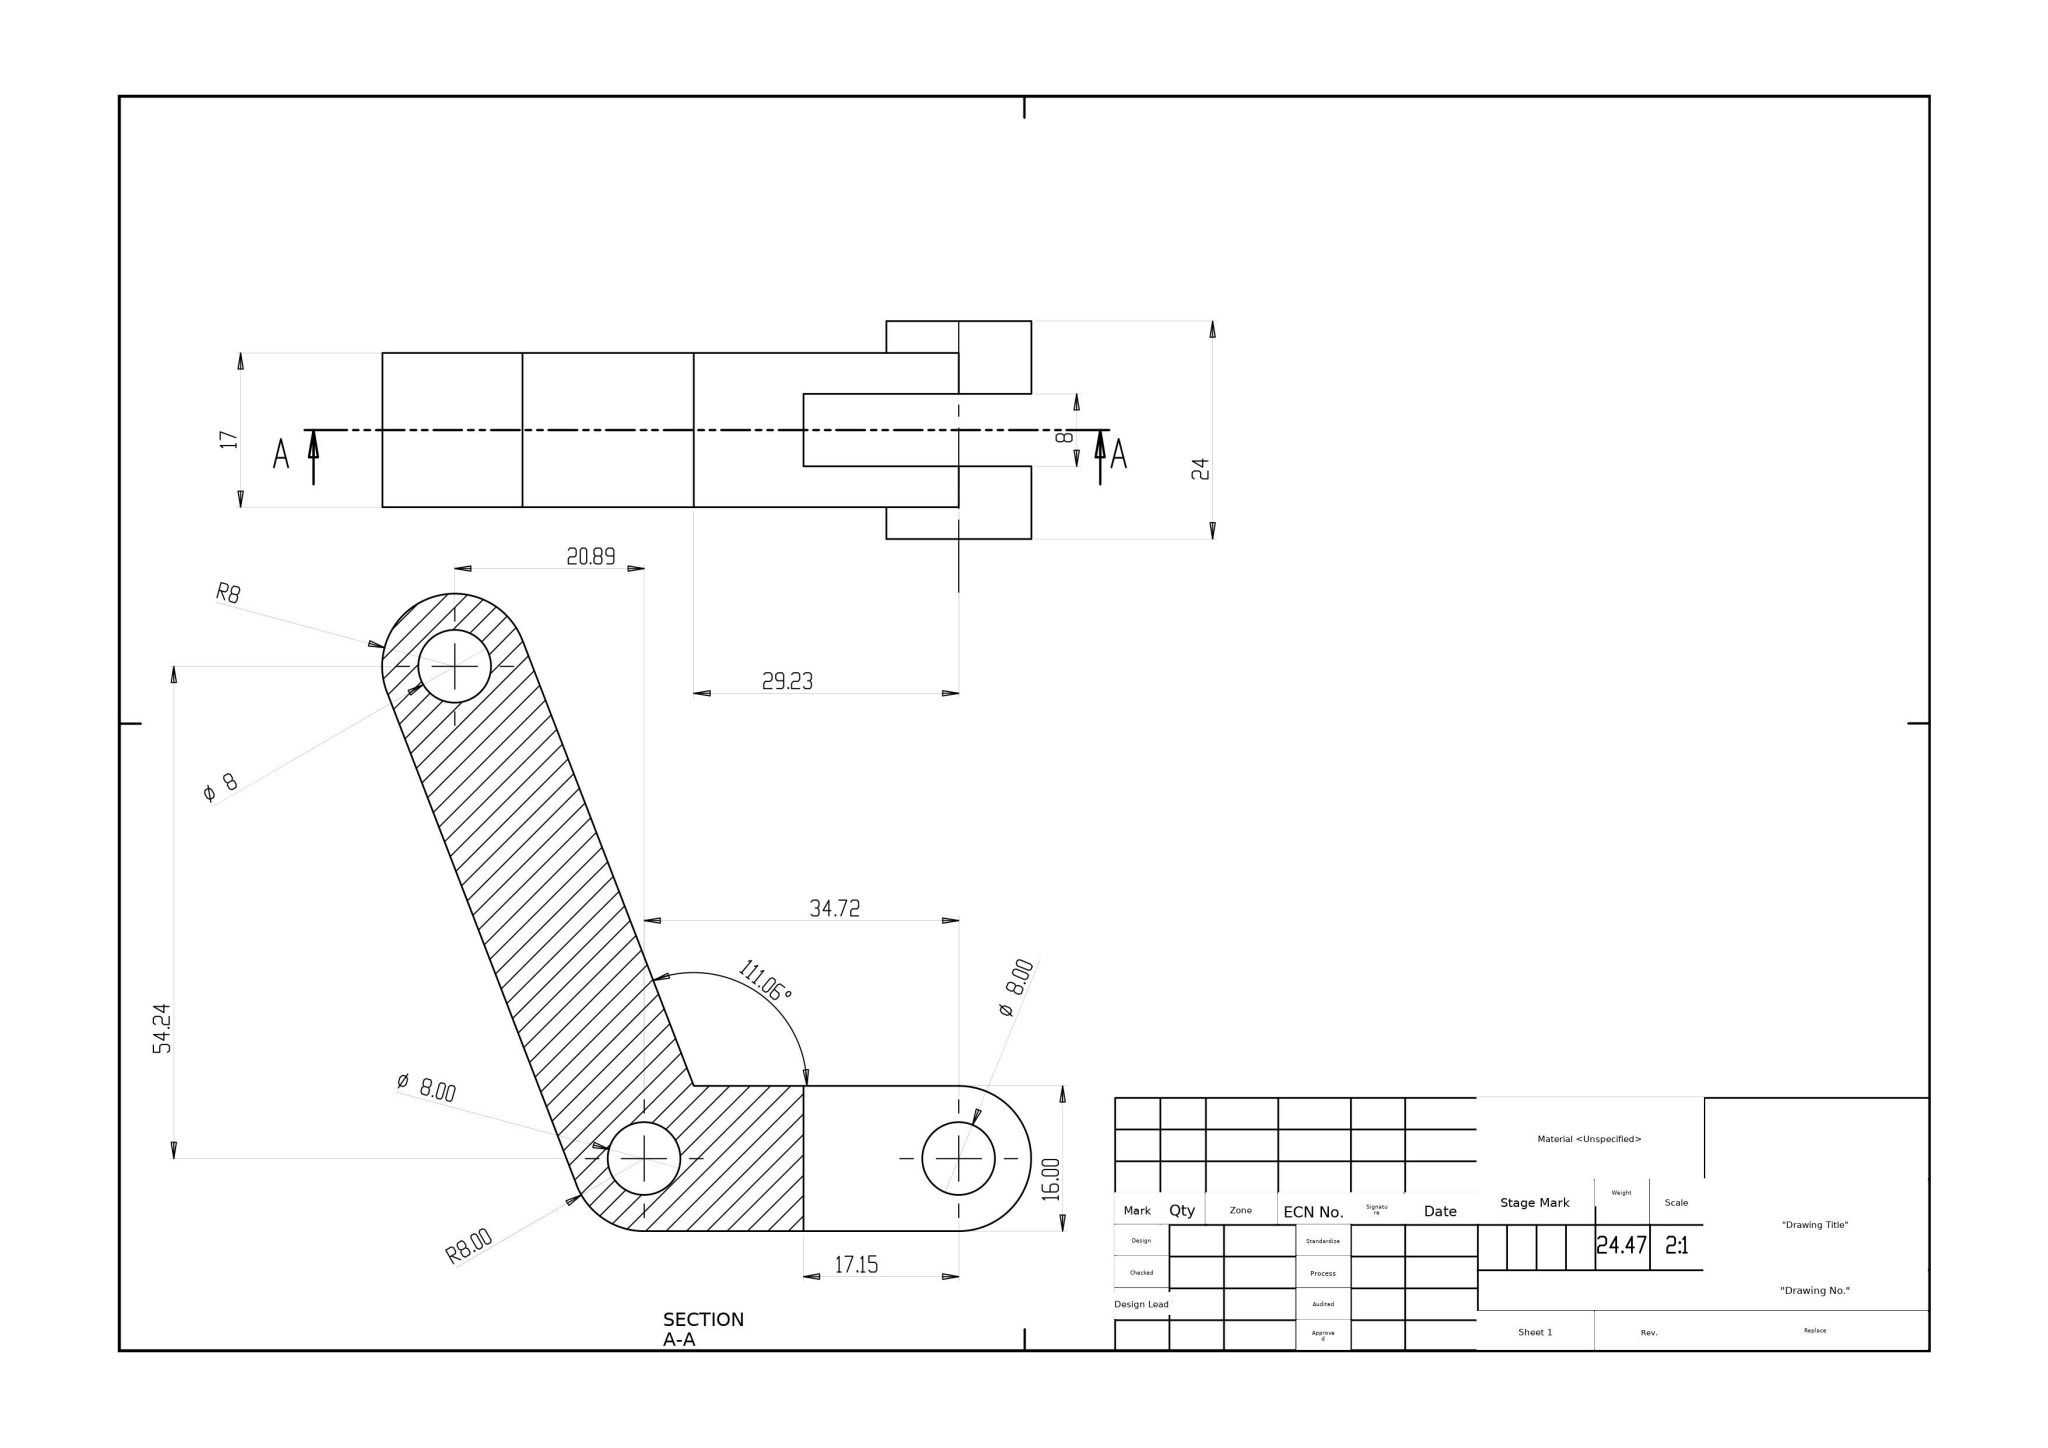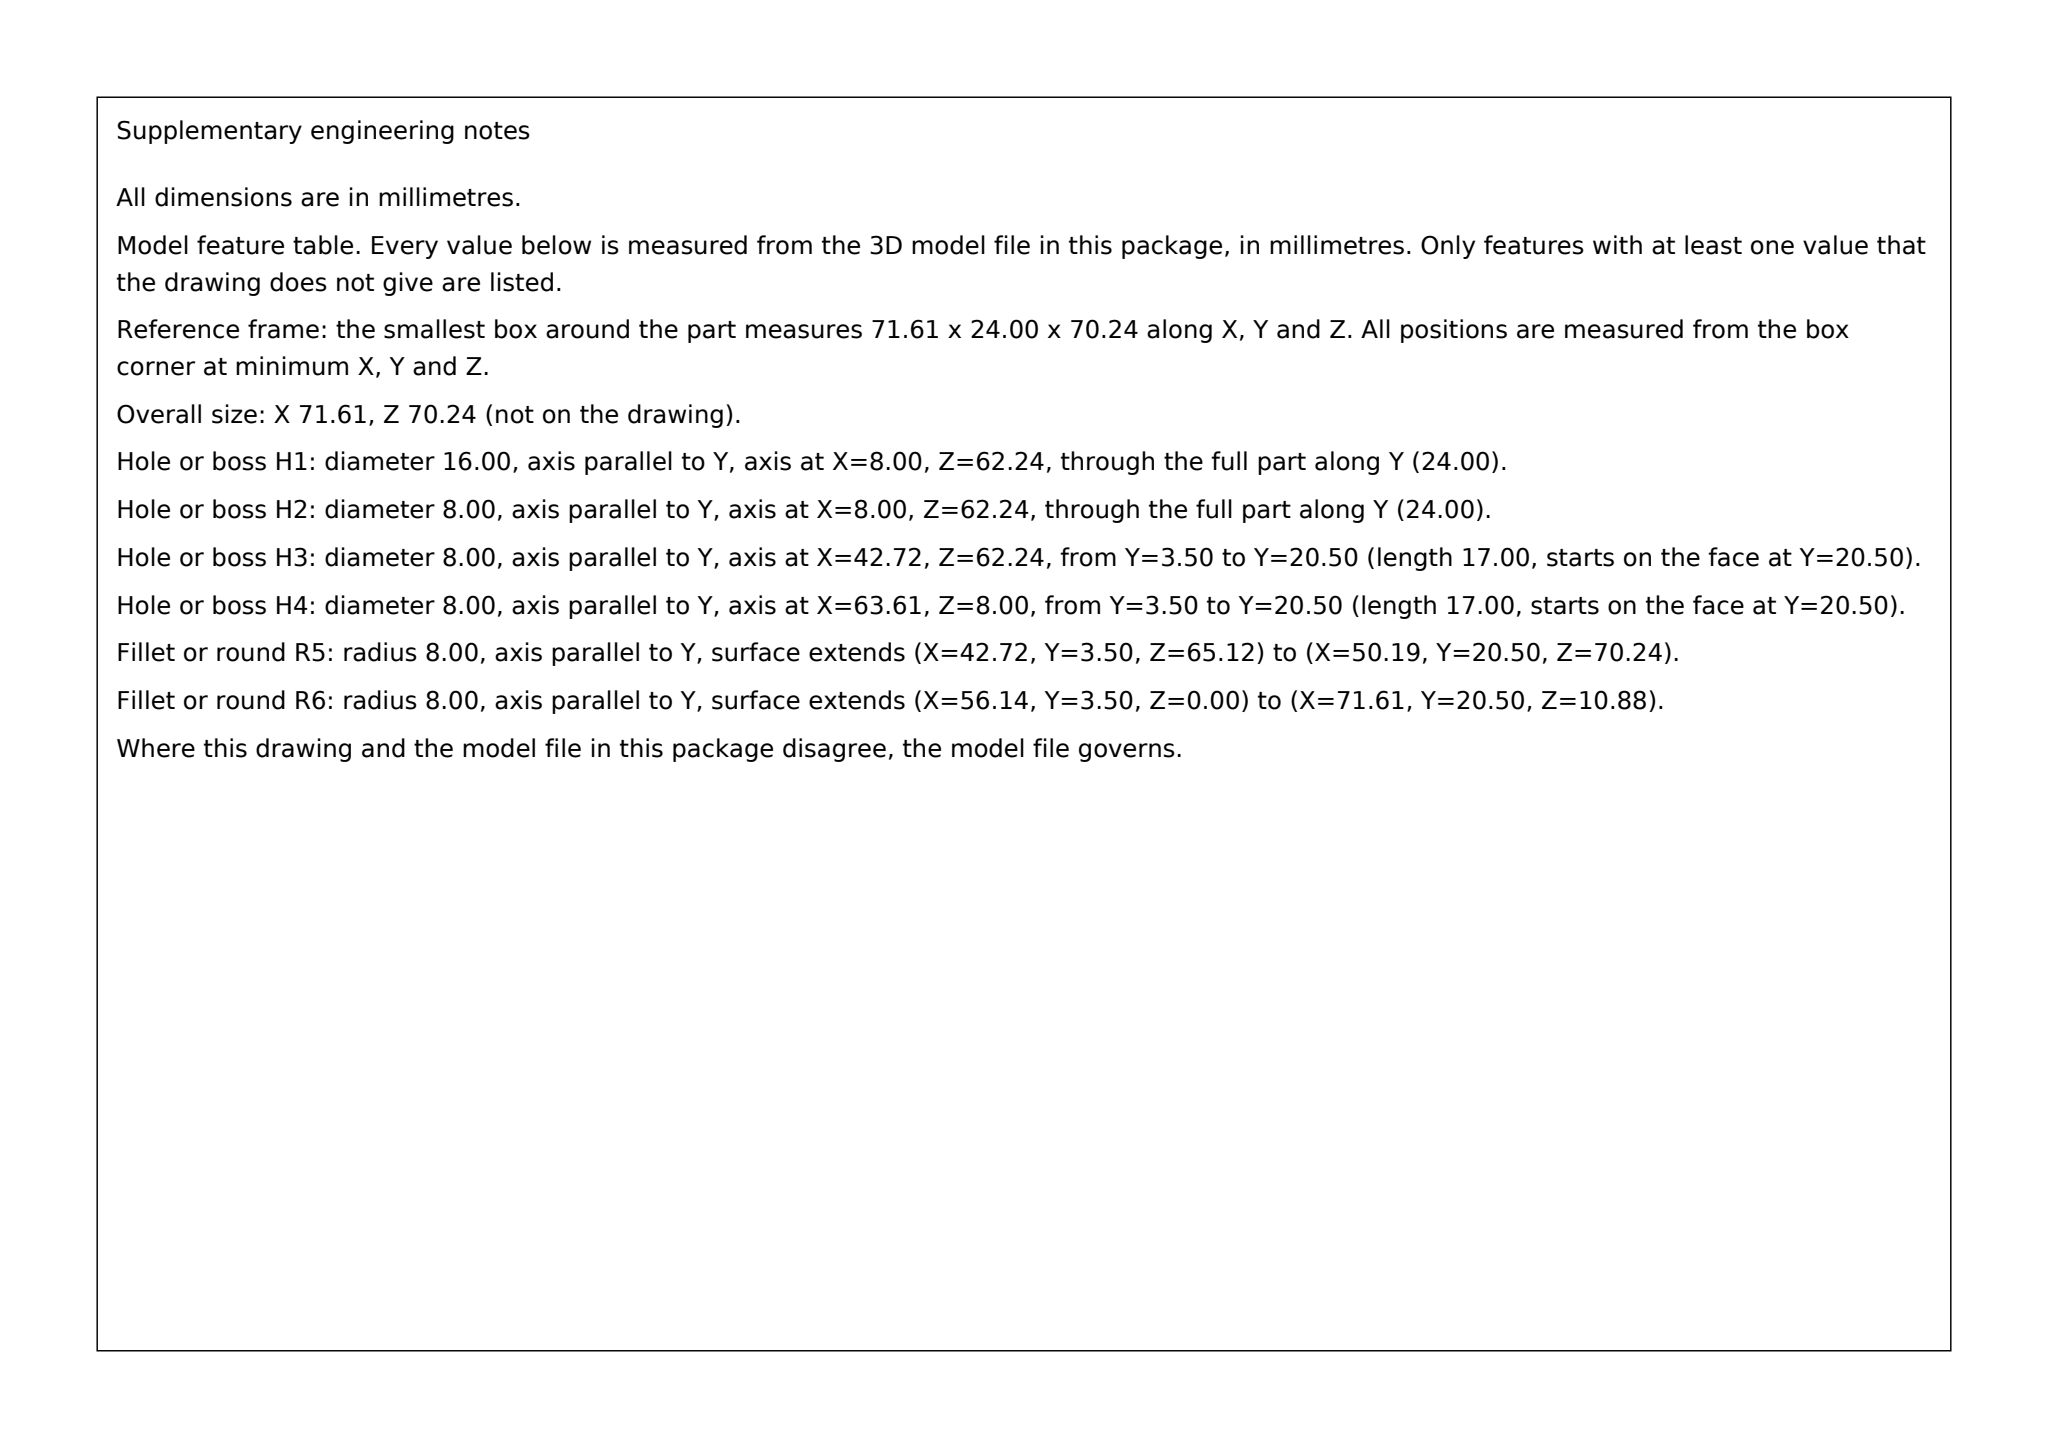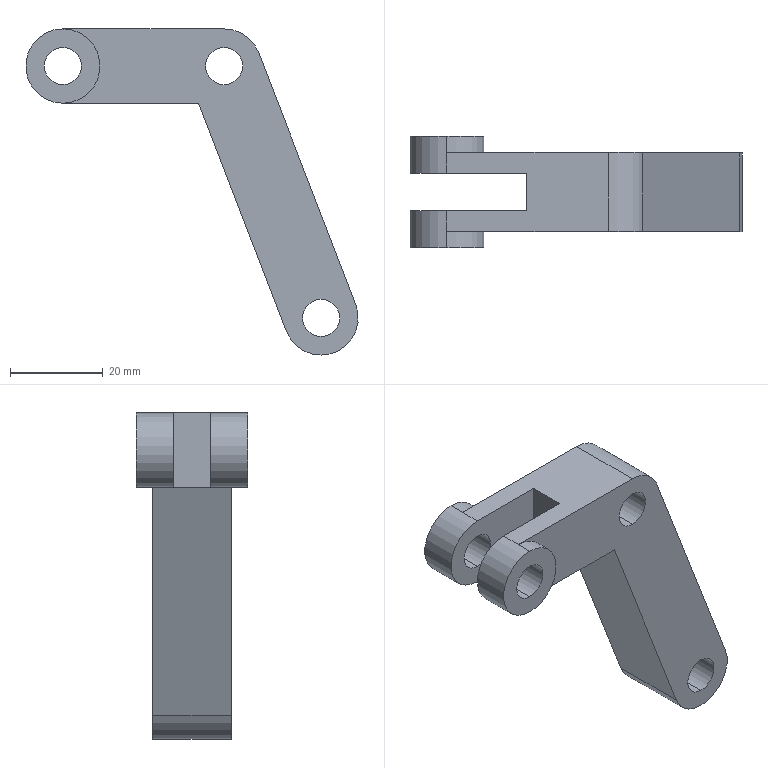Part | SolidWorks | mm | 1 solid | 26 faces | box 71.61 x 24 x 70.24 mm | volume 24474 mm3 | cylinder 15 | plane 11 | commonest cylinder face diameters 8 x8 16 x7
build123d program:
from build123d import *

# Parameters (mm, degrees)
SKETCH1_R           = 4
BOSS_EXTRUDE1_DEPTH = 8.5
SKETCH2_W           = 25.15
SKETCH2_H           = 8
CUT_EXTRUDE1_DEPTH  = 16
SKETCH4_R           = 8
SKETCH4_R_2         = 4
BOSS_EXTRUDE2_DEPTH = 3.5


with BuildPart() as part:
    # Sketch1 → Boss-Extrude1 (new, symmetric)
    with BuildSketch(Plane(origin=(0, 0, 0), x_dir=(1, 0, 0), z_dir=(0, 1, 0))):
        with BuildLine():
            Line((0, 8), (29.228, 8))
            Line((29.228, 8), (48.145, 57.115))
            ThreePointArc((48.145, 57.115), (58.485, 61.705), (63.075, 51.365))
            Line((63.075, 51.365), (42.185, -2.875))
            ThreePointArc((42.185, -2.875), (39.248, -6.596), (34.72, -8))
            Line((34.72, -8), (0, -8))
            ThreePointArc((0, -8), (-8, 0), (0, 8))
        make_face()
        with Locations(Location((0, 0, 0), (0, 0, 270))):
            Circle(SKETCH1_R, mode=Mode.SUBTRACT)
        with Locations(Location((34.72, 0, 0), (0, 0, 270))):
            Circle(SKETCH1_R, mode=Mode.SUBTRACT)
        with Locations(Location((55.61, 54.24, 0), (0, 0, 270))):
            Circle(SKETCH1_R, mode=Mode.SUBTRACT)
    extrude(amount=BOSS_EXTRUDE1_DEPTH, both=True)

    # Sketch2 → Cut-Extrude1 (cut)
    with BuildSketch(Plane.XY.offset(8)):
        with Locations((4.575, 0)):
            Rectangle(SKETCH2_W, SKETCH2_H)
    extrude(amount=-CUT_EXTRUDE1_DEPTH, mode=Mode.SUBTRACT)

    # Sketch4 → Boss-Extrude2 (add)
    with BuildSketch(Plane.XZ.offset(8.5)):
        with Locations(Location((0, 0, 0), (0, 0, 270))):
            Circle(SKETCH4_R)
        with Locations(Location((0, 0, 0), (0, 0, 90))):
            Circle(SKETCH4_R_2, mode=Mode.SUBTRACT)
    boss_extrude2 = extrude(amount=BOSS_EXTRUDE2_DEPTH)

    # Mirror1: Boss-Extrude2 across plane
    add(boss_extrude2.mirror(Plane.ZX))


solid = part.part
STEP:
#1=CARTESIAN_POINT('',(55.61,8.5,-58.24));
#2=VERTEX_POINT('',#1);
#3=CARTESIAN_POINT('',(55.61,8.5,-50.24));
#4=VERTEX_POINT('',#3);
#5=CARTESIAN_POINT('',(55.61,8.5,-54.24));
#6=DIRECTION('',(0.,1.,0.));
#7=DIRECTION('',(0.,0.,1.));
#8=AXIS2_PLACEMENT_3D('',#5,#6,#7);
#9=CIRCLE('',#8,4.);
#10=EDGE_CURVE('',#2,#4,#9,.T.);
#11=ORIENTED_EDGE('',*,*,#10,.T.);
#12=CARTESIAN_POINT('',(55.61,-8.5,-50.24));
#13=VERTEX_POINT('',#12);
#14=CARTESIAN_POINT('',(55.61,8.5,-50.24));
#15=DIRECTION('',(0.,-1.,0.));
#16=VECTOR('',#15,1000.);
#17=LINE('',#14,#16);
#18=EDGE_CURVE('',#4,#13,#17,.T.);
#19=ORIENTED_EDGE('',*,*,#18,.T.);
#20=CARTESIAN_POINT('',(55.61,-8.5,-58.24));
#21=VERTEX_POINT('',#20);
#22=CARTESIAN_POINT('',(55.61,-8.5,-54.24));
#23=DIRECTION('',(0.,1.,0.));
#24=DIRECTION('',(0.,0.,1.));
#25=AXIS2_PLACEMENT_3D('',#22,#23,#24);
#26=CIRCLE('',#25,4.);
#27=EDGE_CURVE('',#21,#13,#26,.T.);
#28=ORIENTED_EDGE('',*,*,#27,.F.);
#29=CARTESIAN_POINT('',(55.61,8.5,-58.24));
#30=DIRECTION('',(0.,-1.,0.));
#31=VECTOR('',#30,1000.);
#32=LINE('',#29,#31);
#33=EDGE_CURVE('',#2,#21,#32,.T.);
#34=ORIENTED_EDGE('',*,*,#33,.F.);
#35=EDGE_LOOP('',(#11,#19,#28,#34));
#36=FACE_OUTER_BOUND('',#35,.T.);
#37=CARTESIAN_POINT('',(55.61,8.5,-54.24));
#38=DIRECTION('',(0.,-1.,0.));
#39=DIRECTION('',(0.,0.,-1.));
#40=AXIS2_PLACEMENT_3D('',#37,#38,#39);
#41=CYLINDRICAL_SURFACE('',#40,4.);
#42=ADVANCED_FACE('',(#36),#41,.F.);
#43=CARTESIAN_POINT('',(34.72,8.5,-4.));
#44=VERTEX_POINT('',#43);
#45=CARTESIAN_POINT('',(34.72,8.5,4.));
#46=VERTEX_POINT('',#45);
#47=CARTESIAN_POINT('',(34.72,8.5,0.));
#48=DIRECTION('',(0.,1.,0.));
#49=DIRECTION('',(0.,0.,1.));
#50=AXIS2_PLACEMENT_3D('',#47,#48,#49);
#51=CIRCLE('',#50,4.);
#52=EDGE_CURVE('',#44,#46,#51,.T.);
#53=ORIENTED_EDGE('',*,*,#52,.T.);
#54=CARTESIAN_POINT('',(34.72,-8.5,4.));
#55=VERTEX_POINT('',#54);
#56=CARTESIAN_POINT('',(34.72,8.5,4.));
#57=DIRECTION('',(0.,-1.,0.));
#58=VECTOR('',#57,1000.);
#59=LINE('',#56,#58);
#60=EDGE_CURVE('',#46,#55,#59,.T.);
#61=ORIENTED_EDGE('',*,*,#60,.T.);
#62=CARTESIAN_POINT('',(34.72,-8.5,-4.));
#63=VERTEX_POINT('',#62);
#64=CARTESIAN_POINT('',(34.72,-8.5,0.));
#65=DIRECTION('',(0.,1.,0.));
#66=DIRECTION('',(0.,0.,1.));
#67=AXIS2_PLACEMENT_3D('',#64,#65,#66);
#68=CIRCLE('',#67,4.);
#69=EDGE_CURVE('',#63,#55,#68,.T.);
#70=ORIENTED_EDGE('',*,*,#69,.F.);
#71=CARTESIAN_POINT('',(34.72,8.5,-4.));
#72=DIRECTION('',(0.,-1.,0.));
#73=VECTOR('',#72,1000.);
#74=LINE('',#71,#73);
#75=EDGE_CURVE('',#44,#63,#74,.T.);
#76=ORIENTED_EDGE('',*,*,#75,.F.);
#77=EDGE_LOOP('',(#53,#61,#70,#76));
#78=FACE_OUTER_BOUND('',#77,.T.);
#79=CARTESIAN_POINT('',(34.72,8.5,0.));
#80=DIRECTION('',(0.,-1.,0.));
#81=DIRECTION('',(0.,0.,-1.));
#82=AXIS2_PLACEMENT_3D('',#79,#80,#81);
#83=CYLINDRICAL_SURFACE('',#82,4.);
#84=ADVANCED_FACE('',(#78),#83,.F.);
#85=CARTESIAN_POINT('',(0.,-4.,-4.));
#86=VERTEX_POINT('',#85);
#87=CARTESIAN_POINT('',(0.,-4.,4.));
#88=VERTEX_POINT('',#87);
#89=CARTESIAN_POINT('',(0.,-4.,0.));
#90=DIRECTION('',(0.,1.,0.));
#91=DIRECTION('',(0.,0.,-1.));
#92=AXIS2_PLACEMENT_3D('',#89,#90,#91);
#93=CIRCLE('',#92,4.);
#94=EDGE_CURVE('',#86,#88,#93,.T.);
#95=ORIENTED_EDGE('',*,*,#94,.T.);
#96=CARTESIAN_POINT('',(0.,-12.,4.));
#97=VERTEX_POINT('',#96);
#98=CARTESIAN_POINT('',(0.,8.5,4.));
#99=DIRECTION('',(0.,-1.,0.));
#100=VECTOR('',#99,1000.);
#101=LINE('',#98,#100);
#102=EDGE_CURVE('',#88,#97,#101,.T.);
#103=ORIENTED_EDGE('',*,*,#102,.T.);
#104=CARTESIAN_POINT('',(0.,-12.,-4.));
#105=VERTEX_POINT('',#104);
#106=CARTESIAN_POINT('',(0.,-12.,0.));
#107=DIRECTION('',(0.,-1.,0.));
#108=DIRECTION('',(0.,0.,-1.));
#109=AXIS2_PLACEMENT_3D('',#106,#107,#108);
#110=CIRCLE('',#109,4.);
#111=EDGE_CURVE('',#97,#105,#110,.T.);
#112=ORIENTED_EDGE('',*,*,#111,.T.);
#113=CARTESIAN_POINT('',(0.,8.5,-4.));
#114=DIRECTION('',(0.,-1.,0.));
#115=VECTOR('',#114,1000.);
#116=LINE('',#113,#115);
#117=EDGE_CURVE('',#86,#105,#116,.T.);
#118=ORIENTED_EDGE('',*,*,#117,.F.);
#119=EDGE_LOOP('',(#95,#103,#112,#118));
#120=FACE_OUTER_BOUND('',#119,.T.);
#121=CARTESIAN_POINT('',(0.,8.5,0.));
#122=DIRECTION('',(0.,-1.,0.));
#123=DIRECTION('',(0.,0.,-1.));
#124=AXIS2_PLACEMENT_3D('',#121,#122,#123);
#125=CYLINDRICAL_SURFACE('',#124,4.);
#126=ADVANCED_FACE('',(#120),#125,.F.);
#127=CARTESIAN_POINT('',(55.61,8.5,-62.24));
#128=VERTEX_POINT('',#127);
#129=CARTESIAN_POINT('',(48.145,8.5,-57.115));
#130=VERTEX_POINT('',#129);
#131=CARTESIAN_POINT('',(55.61,8.5,-54.24));
#132=DIRECTION('',(0.,1.,0.));
#133=DIRECTION('',(0.,0.,-1.));
#134=AXIS2_PLACEMENT_3D('',#131,#132,#133);
#135=CIRCLE('',#134,8.);
#136=EDGE_CURVE('',#128,#130,#135,.T.);
#137=ORIENTED_EDGE('',*,*,#136,.F.);
#138=CARTESIAN_POINT('',(55.61,-8.5,-62.24));
#139=VERTEX_POINT('',#138);
#140=CARTESIAN_POINT('',(55.61,8.5,-62.24));
#141=DIRECTION('',(0.,-1.,0.));
#142=VECTOR('',#141,1000.);
#143=LINE('',#140,#142);
#144=EDGE_CURVE('',#128,#139,#143,.T.);
#145=ORIENTED_EDGE('',*,*,#144,.T.);
#146=CARTESIAN_POINT('',(48.145,-8.5,-57.115));
#147=VERTEX_POINT('',#146);
#148=CARTESIAN_POINT('',(55.61,-8.5,-54.24));
#149=DIRECTION('',(0.,1.,0.));
#150=DIRECTION('',(0.,0.,-1.));
#151=AXIS2_PLACEMENT_3D('',#148,#149,#150);
#152=CIRCLE('',#151,8.);
#153=EDGE_CURVE('',#139,#147,#152,.T.);
#154=ORIENTED_EDGE('',*,*,#153,.T.);
#155=CARTESIAN_POINT('',(48.145,8.5,-57.115));
#156=DIRECTION('',(0.,-1.,0.));
#157=VECTOR('',#156,1000.);
#158=LINE('',#155,#157);
#159=EDGE_CURVE('',#130,#147,#158,.T.);
#160=ORIENTED_EDGE('',*,*,#159,.F.);
#161=EDGE_LOOP('',(#137,#145,#154,#160));
#162=FACE_OUTER_BOUND('',#161,.T.);
#163=CARTESIAN_POINT('',(55.61,8.5,-54.24));
#164=DIRECTION('',(0.,-1.,0.));
#165=DIRECTION('',(0.,0.,-1.));
#166=AXIS2_PLACEMENT_3D('',#163,#164,#165);
#167=CYLINDRICAL_SURFACE('',#166,8.);
#168=ADVANCED_FACE('',(#162),#167,.T.);
#169=CARTESIAN_POINT('',(0.,-8.5,-8.));
#170=VERTEX_POINT('',#169);
#171=CARTESIAN_POINT('',(0.,-8.5,8.));
#172=VERTEX_POINT('',#171);
#173=CARTESIAN_POINT('',(0.,-8.5,0.));
#174=DIRECTION('',(0.,-1.,0.));
#175=DIRECTION('',(0.,0.,-1.));
#176=AXIS2_PLACEMENT_3D('',#173,#174,#175);
#177=CIRCLE('',#176,8.);
#178=EDGE_CURVE('',#170,#172,#177,.T.);
#179=ORIENTED_EDGE('',*,*,#178,.T.);
#180=CARTESIAN_POINT('',(0.,-12.,8.));
#181=VERTEX_POINT('',#180);
#182=CARTESIAN_POINT('',(0.,8.5,8.));
#183=DIRECTION('',(0.,-1.,0.));
#184=VECTOR('',#183,1000.);
#185=LINE('',#182,#184);
#186=EDGE_CURVE('',#172,#181,#185,.T.);
#187=ORIENTED_EDGE('',*,*,#186,.T.);
#188=CARTESIAN_POINT('',(0.,-12.,-8.));
#189=VERTEX_POINT('',#188);
#190=CARTESIAN_POINT('',(0.,-12.,0.));
#191=DIRECTION('',(0.,-1.,0.));
#192=DIRECTION('',(0.,0.,-1.));
#193=AXIS2_PLACEMENT_3D('',#190,#191,#192);
#194=CIRCLE('',#193,8.);
#195=EDGE_CURVE('',#189,#181,#194,.T.);
#196=ORIENTED_EDGE('',*,*,#195,.F.);
#197=CARTESIAN_POINT('',(0.,8.5,-8.));
#198=DIRECTION('',(0.,-1.,0.));
#199=VECTOR('',#198,1000.);
#200=LINE('',#197,#199);
#201=EDGE_CURVE('',#170,#189,#200,.T.);
#202=ORIENTED_EDGE('',*,*,#201,.F.);
#203=EDGE_LOOP('',(#179,#187,#196,#202));
#204=FACE_OUTER_BOUND('',#203,.T.);
#205=CARTESIAN_POINT('',(0.,8.5,0.));
#206=DIRECTION('',(0.,-1.,0.));
#207=DIRECTION('',(0.,0.,-1.));
#208=AXIS2_PLACEMENT_3D('',#205,#206,#207);
#209=CYLINDRICAL_SURFACE('',#208,8.);
#210=ADVANCED_FACE('',(#204),#209,.T.);
#211=CARTESIAN_POINT('',(0.,12.,4.));
#212=VERTEX_POINT('',#211);
#213=CARTESIAN_POINT('',(0.,12.,-4.));
#214=VERTEX_POINT('',#213);
#215=CARTESIAN_POINT('',(0.,12.,0.));
#216=DIRECTION('',(0.,-1.,0.));
#217=DIRECTION('',(0.,0.,-1.));
#218=AXIS2_PLACEMENT_3D('',#215,#216,#217);
#219=CIRCLE('',#218,4.);
#220=EDGE_CURVE('',#212,#214,#219,.T.);
#221=ORIENTED_EDGE('',*,*,#220,.F.);
#222=CARTESIAN_POINT('',(0.,4.,4.));
#223=VERTEX_POINT('',#222);
#224=CARTESIAN_POINT('',(0.,8.5,4.));
#225=DIRECTION('',(0.,-1.,0.));
#226=VECTOR('',#225,1000.);
#227=LINE('',#224,#226);
#228=EDGE_CURVE('',#212,#223,#227,.T.);
#229=ORIENTED_EDGE('',*,*,#228,.T.);
#230=CARTESIAN_POINT('',(0.,4.,-4.));
#231=VERTEX_POINT('',#230);
#232=CARTESIAN_POINT('',(0.,4.,0.));
#233=DIRECTION('',(0.,-1.,0.));
#234=DIRECTION('',(0.,0.,1.));
#235=AXIS2_PLACEMENT_3D('',#232,#233,#234);
#236=CIRCLE('',#235,4.);
#237=EDGE_CURVE('',#223,#231,#236,.T.);
#238=ORIENTED_EDGE('',*,*,#237,.T.);
#239=CARTESIAN_POINT('',(0.,8.5,-4.));
#240=DIRECTION('',(0.,-1.,0.));
#241=VECTOR('',#240,1000.);
#242=LINE('',#239,#241);
#243=EDGE_CURVE('',#214,#231,#242,.T.);
#244=ORIENTED_EDGE('',*,*,#243,.F.);
#245=EDGE_LOOP('',(#221,#229,#238,#244));
#246=FACE_OUTER_BOUND('',#245,.T.);
#247=CARTESIAN_POINT('',(0.,8.5,0.));
#248=DIRECTION('',(0.,-1.,0.));
#249=DIRECTION('',(0.,0.,-1.));
#250=AXIS2_PLACEMENT_3D('',#247,#248,#249);
#251=CYLINDRICAL_SURFACE('',#250,4.);
#252=ADVANCED_FACE('',(#246),#251,.F.);
#253=CARTESIAN_POINT('',(0.,12.,-8.));
#254=VERTEX_POINT('',#253);
#255=CARTESIAN_POINT('',(0.,12.,8.));
#256=VERTEX_POINT('',#255);
#257=CARTESIAN_POINT('',(0.,12.,0.));
#258=DIRECTION('',(0.,-1.,0.));
#259=DIRECTION('',(0.,0.,-1.));
#260=AXIS2_PLACEMENT_3D('',#257,#258,#259);
#261=CIRCLE('',#260,8.);
#262=EDGE_CURVE('',#254,#256,#261,.T.);
#263=ORIENTED_EDGE('',*,*,#262,.T.);
#264=CARTESIAN_POINT('',(0.,8.5,8.));
#265=VERTEX_POINT('',#264);
#266=CARTESIAN_POINT('',(0.,8.5,8.));
#267=DIRECTION('',(0.,-1.,0.));
#268=VECTOR('',#267,1000.);
#269=LINE('',#266,#268);
#270=EDGE_CURVE('',#256,#265,#269,.T.);
#271=ORIENTED_EDGE('',*,*,#270,.T.);
#272=CARTESIAN_POINT('',(0.,8.5,-8.));
#273=VERTEX_POINT('',#272);
#274=CARTESIAN_POINT('',(0.,8.5,0.));
#275=DIRECTION('',(0.,-1.,0.));
#276=DIRECTION('',(0.,0.,-1.));
#277=AXIS2_PLACEMENT_3D('',#274,#275,#276);
#278=CIRCLE('',#277,8.);
#279=EDGE_CURVE('',#273,#265,#278,.T.);
#280=ORIENTED_EDGE('',*,*,#279,.F.);
#281=CARTESIAN_POINT('',(0.,8.5,-8.));
#282=DIRECTION('',(0.,-1.,0.));
#283=VECTOR('',#282,1000.);
#284=LINE('',#281,#283);
#285=EDGE_CURVE('',#254,#273,#284,.T.);
#286=ORIENTED_EDGE('',*,*,#285,.F.);
#287=EDGE_LOOP('',(#263,#271,#280,#286));
#288=FACE_OUTER_BOUND('',#287,.T.);
#289=CARTESIAN_POINT('',(0.,8.5,0.));
#290=DIRECTION('',(0.,-1.,0.));
#291=DIRECTION('',(0.,0.,-1.));
#292=AXIS2_PLACEMENT_3D('',#289,#290,#291);
#293=CYLINDRICAL_SURFACE('',#292,8.);
#294=ADVANCED_FACE('',(#288),#293,.T.);
#295=ORIENTED_EDGE('',*,*,#270,.F.);
#296=CARTESIAN_POINT('',(0.,12.,0.));
#297=DIRECTION('',(0.,-1.,0.));
#298=DIRECTION('',(0.,0.,-1.));
#299=AXIS2_PLACEMENT_3D('',#296,#297,#298);
#300=CIRCLE('',#299,8.);
#301=EDGE_CURVE('',#256,#254,#300,.T.);
#302=ORIENTED_EDGE('',*,*,#301,.T.);
#303=ORIENTED_EDGE('',*,*,#285,.T.);
#304=CARTESIAN_POINT('',(0.,4.,-8.));
#305=VERTEX_POINT('',#304);
#306=CARTESIAN_POINT('',(0.,8.5,-8.));
#307=DIRECTION('',(0.,-1.,0.));
#308=VECTOR('',#307,1000.);
#309=LINE('',#306,#308);
#310=EDGE_CURVE('',#273,#305,#309,.T.);
#311=ORIENTED_EDGE('',*,*,#310,.T.);
#312=CARTESIAN_POINT('',(0.,4.,8.));
#313=VERTEX_POINT('',#312);
#314=CARTESIAN_POINT('',(0.,4.,0.));
#315=DIRECTION('',(0.,-1.,0.));
#316=DIRECTION('',(0.,0.,1.));
#317=AXIS2_PLACEMENT_3D('',#314,#315,#316);
#318=CIRCLE('',#317,8.);
#319=EDGE_CURVE('',#313,#305,#318,.T.);
#320=ORIENTED_EDGE('',*,*,#319,.F.);
#321=CARTESIAN_POINT('',(0.,8.5,8.));
#322=DIRECTION('',(0.,-1.,0.));
#323=VECTOR('',#322,1000.);
#324=LINE('',#321,#323);
#325=EDGE_CURVE('',#265,#313,#324,.T.);
#326=ORIENTED_EDGE('',*,*,#325,.F.);
#327=EDGE_LOOP('',(#295,#302,#303,#311,#320,#326));
#328=FACE_OUTER_BOUND('',#327,.T.);
#329=CARTESIAN_POINT('',(0.,8.5,0.));
#330=DIRECTION('',(0.,-1.,0.));
#331=DIRECTION('',(0.,0.,-1.));
#332=AXIS2_PLACEMENT_3D('',#329,#330,#331);
#333=CYLINDRICAL_SURFACE('',#332,8.);
#334=ADVANCED_FACE('',(#328),#333,.T.);
#335=ORIENTED_EDGE('',*,*,#228,.F.);
#336=CARTESIAN_POINT('',(0.,12.,0.));
#337=DIRECTION('',(0.,-1.,0.));
#338=DIRECTION('',(0.,0.,-1.));
#339=AXIS2_PLACEMENT_3D('',#336,#337,#338);
#340=CIRCLE('',#339,4.);
#341=EDGE_CURVE('',#214,#212,#340,.T.);
#342=ORIENTED_EDGE('',*,*,#341,.F.);
#343=ORIENTED_EDGE('',*,*,#243,.T.);
#344=CARTESIAN_POINT('',(0.,4.,0.));
#345=DIRECTION('',(0.,-1.,0.));
#346=DIRECTION('',(0.,0.,1.));
#347=AXIS2_PLACEMENT_3D('',#344,#345,#346);
#348=CIRCLE('',#347,4.);
#349=EDGE_CURVE('',#231,#223,#348,.T.);
#350=ORIENTED_EDGE('',*,*,#349,.T.);
#351=EDGE_LOOP('',(#335,#342,#343,#350));
#352=FACE_OUTER_BOUND('',#351,.T.);
#353=CARTESIAN_POINT('',(0.,8.5,0.));
#354=DIRECTION('',(0.,-1.,0.));
#355=DIRECTION('',(0.,0.,-1.));
#356=AXIS2_PLACEMENT_3D('',#353,#354,#355);
#357=CYLINDRICAL_SURFACE('',#356,4.);
#358=ADVANCED_FACE('',(#352),#357,.F.);
#359=CARTESIAN_POINT('',(29.228,8.5,-8.));
#360=VERTEX_POINT('',#359);
#361=CARTESIAN_POINT('',(0.,8.5,-8.));
#362=DIRECTION('',(-1.,0.,0.));
#363=VECTOR('',#362,1000.);
#364=LINE('',#361,#363);
#365=EDGE_CURVE('',#360,#273,#364,.T.);
#366=ORIENTED_EDGE('',*,*,#365,.T.);
#367=ORIENTED_EDGE('',*,*,#279,.T.);
#368=CARTESIAN_POINT('',(34.72,8.5,8.));
#369=VERTEX_POINT('',#368);
#370=CARTESIAN_POINT('',(34.72,8.5,8.));
#371=DIRECTION('',(1.,0.,-0.));
#372=VECTOR('',#371,1000.);
#373=LINE('',#370,#372);
#374=EDGE_CURVE('',#265,#369,#373,.T.);
#375=ORIENTED_EDGE('',*,*,#374,.T.);
#376=CARTESIAN_POINT('',(42.185,8.5,2.875));
#377=VERTEX_POINT('',#376);
#378=CARTESIAN_POINT('',(34.72,8.5,-0.));
#379=DIRECTION('',(0.,1.,0.));
#380=DIRECTION('',(0.,0.,-1.));
#381=AXIS2_PLACEMENT_3D('',#378,#379,#380);
#382=CIRCLE('',#381,8.);
#383=EDGE_CURVE('',#369,#377,#382,.T.);
#384=ORIENTED_EDGE('',*,*,#383,.T.);
#385=CARTESIAN_POINT('',(63.075,8.5,-51.365));
#386=VERTEX_POINT('',#385);
#387=CARTESIAN_POINT('',(63.075,8.5,-51.365));
#388=DIRECTION('',(0.3594,0.,-0.9332));
#389=VECTOR('',#388,1000.);
#390=LINE('',#387,#389);
#391=EDGE_CURVE('',#377,#386,#390,.T.);
#392=ORIENTED_EDGE('',*,*,#391,.T.);
#393=CARTESIAN_POINT('',(55.61,8.5,-54.24));
#394=DIRECTION('',(0.,1.,0.));
#395=DIRECTION('',(0.,0.,-1.));
#396=AXIS2_PLACEMENT_3D('',#393,#394,#395);
#397=CIRCLE('',#396,8.);
#398=EDGE_CURVE('',#386,#128,#397,.T.);
#399=ORIENTED_EDGE('',*,*,#398,.T.);
#400=ORIENTED_EDGE('',*,*,#136,.T.);
#401=CARTESIAN_POINT('',(29.228,8.5,-8.));
#402=DIRECTION('',(-0.3594,0.,0.9332));
#403=VECTOR('',#402,1000.);
#404=LINE('',#401,#403);
#405=EDGE_CURVE('',#130,#360,#404,.T.);
#406=ORIENTED_EDGE('',*,*,#405,.T.);
#407=EDGE_LOOP('',(#366,#367,#375,#384,#392,#399,#400,#406));
#408=FACE_OUTER_BOUND('',#407,.T.);
#409=ORIENTED_EDGE('',*,*,#52,.F.);
#410=CARTESIAN_POINT('',(34.72,8.5,0.));
#411=DIRECTION('',(0.,1.,0.));
#412=DIRECTION('',(0.,0.,1.));
#413=AXIS2_PLACEMENT_3D('',#410,#411,#412);
#414=CIRCLE('',#413,4.);
#415=EDGE_CURVE('',#46,#44,#414,.T.);
#416=ORIENTED_EDGE('',*,*,#415,.F.);
#417=EDGE_LOOP('',(#409,#416));
#418=FACE_BOUND('',#417,.T.);
#419=ORIENTED_EDGE('',*,*,#10,.F.);
#420=CARTESIAN_POINT('',(55.61,8.5,-54.24));
#421=DIRECTION('',(0.,1.,0.));
#422=DIRECTION('',(0.,0.,1.));
#423=AXIS2_PLACEMENT_3D('',#420,#421,#422);
#424=CIRCLE('',#423,4.);
#425=EDGE_CURVE('',#4,#2,#424,.T.);
#426=ORIENTED_EDGE('',*,*,#425,.F.);
#427=EDGE_LOOP('',(#419,#426));
#428=FACE_BOUND('',#427,.T.);
#429=CARTESIAN_POINT('',(0.,8.5,0.));
#430=DIRECTION('',(0.,-1.,0.));
#431=DIRECTION('',(0.,0.,-1.));
#432=AXIS2_PLACEMENT_3D('',#429,#430,#431);
#433=PLANE('',#432);
#434=ADVANCED_FACE('',(#408,#418,#428),#433,.F.);
#435=ORIENTED_EDGE('',*,*,#178,.F.);
#436=CARTESIAN_POINT('',(29.228,-8.5,-8.));
#437=VERTEX_POINT('',#436);
#438=CARTESIAN_POINT('',(0.,-8.5,-8.));
#439=DIRECTION('',(-1.,0.,0.));
#440=VECTOR('',#439,1000.);
#441=LINE('',#438,#440);
#442=EDGE_CURVE('',#437,#170,#441,.T.);
#443=ORIENTED_EDGE('',*,*,#442,.F.);
#444=CARTESIAN_POINT('',(29.228,-8.5,-8.));
#445=DIRECTION('',(-0.3594,0.,0.9332));
#446=VECTOR('',#445,1000.);
#447=LINE('',#444,#446);
#448=EDGE_CURVE('',#147,#437,#447,.T.);
#449=ORIENTED_EDGE('',*,*,#448,.F.);
#450=ORIENTED_EDGE('',*,*,#153,.F.);
#451=CARTESIAN_POINT('',(63.075,-8.5,-51.365));
#452=VERTEX_POINT('',#451);
#453=CARTESIAN_POINT('',(55.61,-8.5,-54.24));
#454=DIRECTION('',(0.,1.,0.));
#455=DIRECTION('',(0.,0.,-1.));
#456=AXIS2_PLACEMENT_3D('',#453,#454,#455);
#457=CIRCLE('',#456,8.);
#458=EDGE_CURVE('',#452,#139,#457,.T.);
#459=ORIENTED_EDGE('',*,*,#458,.F.);
#460=CARTESIAN_POINT('',(42.185,-8.5,2.875));
#461=VERTEX_POINT('',#460);
#462=CARTESIAN_POINT('',(63.075,-8.5,-51.365));
#463=DIRECTION('',(0.3594,0.,-0.9332));
#464=VECTOR('',#463,1000.);
#465=LINE('',#462,#464);
#466=EDGE_CURVE('',#461,#452,#465,.T.);
#467=ORIENTED_EDGE('',*,*,#466,.F.);
#468=CARTESIAN_POINT('',(34.72,-8.5,8.));
#469=VERTEX_POINT('',#468);
#470=CARTESIAN_POINT('',(34.72,-8.5,-0.));
#471=DIRECTION('',(0.,1.,0.));
#472=DIRECTION('',(0.,0.,-1.));
#473=AXIS2_PLACEMENT_3D('',#470,#471,#472);
#474=CIRCLE('',#473,8.);
#475=EDGE_CURVE('',#469,#461,#474,.T.);
#476=ORIENTED_EDGE('',*,*,#475,.F.);
#477=CARTESIAN_POINT('',(34.72,-8.5,8.));
#478=DIRECTION('',(1.,0.,-0.));
#479=VECTOR('',#478,1000.);
#480=LINE('',#477,#479);
#481=EDGE_CURVE('',#172,#469,#480,.T.);
#482=ORIENTED_EDGE('',*,*,#481,.F.);
#483=EDGE_LOOP('',(#435,#443,#449,#450,#459,#467,#476,#482));
#484=FACE_OUTER_BOUND('',#483,.T.);
#485=ORIENTED_EDGE('',*,*,#69,.T.);
#486=CARTESIAN_POINT('',(34.72,-8.5,0.));
#487=DIRECTION('',(0.,1.,0.));
#488=DIRECTION('',(0.,0.,1.));
#489=AXIS2_PLACEMENT_3D('',#486,#487,#488);
#490=CIRCLE('',#489,4.);
#491=EDGE_CURVE('',#55,#63,#490,.T.);
#492=ORIENTED_EDGE('',*,*,#491,.T.);
#493=EDGE_LOOP('',(#485,#492));
#494=FACE_BOUND('',#493,.T.);
#495=ORIENTED_EDGE('',*,*,#27,.T.);
#496=CARTESIAN_POINT('',(55.61,-8.5,-54.24));
#497=DIRECTION('',(0.,1.,0.));
#498=DIRECTION('',(0.,0.,1.));
#499=AXIS2_PLACEMENT_3D('',#496,#497,#498);
#500=CIRCLE('',#499,4.);
#501=EDGE_CURVE('',#13,#21,#500,.T.);
#502=ORIENTED_EDGE('',*,*,#501,.T.);
#503=EDGE_LOOP('',(#495,#502));
#504=FACE_BOUND('',#503,.T.);
#505=CARTESIAN_POINT('',(0.,-8.5,0.));
#506=DIRECTION('',(0.,-1.,0.));
#507=DIRECTION('',(0.,0.,-1.));
#508=AXIS2_PLACEMENT_3D('',#505,#506,#507);
#509=PLANE('',#508);
#510=ADVANCED_FACE('',(#484,#494,#504),#509,.T.);
#511=ORIENTED_EDGE('',*,*,#186,.F.);
#512=CARTESIAN_POINT('',(-0.,-4.,8.));
#513=VERTEX_POINT('',#512);
#514=CARTESIAN_POINT('',(0.,8.5,8.));
#515=DIRECTION('',(0.,-1.,0.));
#516=VECTOR('',#515,1000.);
#517=LINE('',#514,#516);
#518=EDGE_CURVE('',#513,#172,#517,.T.);
#519=ORIENTED_EDGE('',*,*,#518,.F.);
#520=CARTESIAN_POINT('',(0.,-4.,-8.));
#521=VERTEX_POINT('',#520);
#522=CARTESIAN_POINT('',(0.,-4.,0.));
#523=DIRECTION('',(0.,1.,0.));
#524=DIRECTION('',(0.,0.,-1.));
#525=AXIS2_PLACEMENT_3D('',#522,#523,#524);
#526=CIRCLE('',#525,8.);
#527=EDGE_CURVE('',#521,#513,#526,.T.);
#528=ORIENTED_EDGE('',*,*,#527,.F.);
#529=CARTESIAN_POINT('',(0.,8.5,-8.));
#530=DIRECTION('',(0.,-1.,0.));
#531=VECTOR('',#530,1000.);
#532=LINE('',#529,#531);
#533=EDGE_CURVE('',#521,#170,#532,.T.);
#534=ORIENTED_EDGE('',*,*,#533,.T.);
#535=ORIENTED_EDGE('',*,*,#201,.T.);
#536=CARTESIAN_POINT('',(0.,-12.,0.));
#537=DIRECTION('',(0.,-1.,0.));
#538=DIRECTION('',(0.,0.,-1.));
#539=AXIS2_PLACEMENT_3D('',#536,#537,#538);
#540=CIRCLE('',#539,8.);
#541=EDGE_CURVE('',#181,#189,#540,.T.);
#542=ORIENTED_EDGE('',*,*,#541,.F.);
#543=EDGE_LOOP('',(#511,#519,#528,#534,#535,#542));
#544=FACE_OUTER_BOUND('',#543,.T.);
#545=CARTESIAN_POINT('',(0.,8.5,0.));
#546=DIRECTION('',(0.,-1.,0.));
#547=DIRECTION('',(0.,0.,-1.));
#548=AXIS2_PLACEMENT_3D('',#545,#546,#547);
#549=CYLINDRICAL_SURFACE('',#548,8.);
#550=ADVANCED_FACE('',(#544),#549,.T.);
#551=ORIENTED_EDGE('',*,*,#325,.T.);
#552=CARTESIAN_POINT('',(17.15,4.,8.));
#553=VERTEX_POINT('',#552);
#554=CARTESIAN_POINT('',(-8.,4.,8.));
#555=DIRECTION('',(-1.,0.,0.));
#556=VECTOR('',#555,1000.);
#557=LINE('',#554,#556);
#558=EDGE_CURVE('',#553,#313,#557,.T.);
#559=ORIENTED_EDGE('',*,*,#558,.F.);
#560=CARTESIAN_POINT('',(17.15,-4.,8.));
#561=VERTEX_POINT('',#560);
#562=CARTESIAN_POINT('',(17.15,4.,8.));
#563=DIRECTION('',(0.,1.,0.));
#564=VECTOR('',#563,1000.);
#565=LINE('',#562,#564);
#566=EDGE_CURVE('',#561,#553,#565,.T.);
#567=ORIENTED_EDGE('',*,*,#566,.F.);
#568=CARTESIAN_POINT('',(-8.,-4.,8.));
#569=DIRECTION('',(1.,0.,0.));
#570=VECTOR('',#569,1000.);
#571=LINE('',#568,#570);
#572=EDGE_CURVE('',#513,#561,#571,.T.);
#573=ORIENTED_EDGE('',*,*,#572,.F.);
#574=ORIENTED_EDGE('',*,*,#518,.T.);
#575=ORIENTED_EDGE('',*,*,#481,.T.);
#576=CARTESIAN_POINT('',(34.72,8.5,8.));
#577=DIRECTION('',(0.,-1.,0.));
#578=VECTOR('',#577,1000.);
#579=LINE('',#576,#578);
#580=EDGE_CURVE('',#369,#469,#579,.T.);
#581=ORIENTED_EDGE('',*,*,#580,.F.);
#582=ORIENTED_EDGE('',*,*,#374,.F.);
#583=EDGE_LOOP('',(#551,#559,#567,#573,#574,#575,#581,#582));
#584=FACE_OUTER_BOUND('',#583,.T.);
#585=CARTESIAN_POINT('',(34.72,8.5,8.));
#586=DIRECTION('',(-0.,0.,-1.));
#587=DIRECTION('',(-1.,0.,0.));
#588=AXIS2_PLACEMENT_3D('',#585,#586,#587);
#589=PLANE('',#588);
#590=ADVANCED_FACE('',(#584),#589,.F.);
#591=ORIENTED_EDGE('',*,*,#475,.T.);
#592=CARTESIAN_POINT('',(42.185,8.5,2.875));
#593=DIRECTION('',(0.,-1.,0.));
#594=VECTOR('',#593,1000.);
#595=LINE('',#592,#594);
#596=EDGE_CURVE('',#377,#461,#595,.T.);
#597=ORIENTED_EDGE('',*,*,#596,.F.);
#598=ORIENTED_EDGE('',*,*,#383,.F.);
#599=ORIENTED_EDGE('',*,*,#580,.T.);
#600=EDGE_LOOP('',(#591,#597,#598,#599));
#601=FACE_OUTER_BOUND('',#600,.T.);
#602=CARTESIAN_POINT('',(34.72,8.5,-0.));
#603=DIRECTION('',(0.,-1.,0.));
#604=DIRECTION('',(0.,0.,-1.));
#605=AXIS2_PLACEMENT_3D('',#602,#603,#604);
#606=CYLINDRICAL_SURFACE('',#605,8.);
#607=ADVANCED_FACE('',(#601),#606,.T.);
#608=ORIENTED_EDGE('',*,*,#466,.T.);
#609=CARTESIAN_POINT('',(63.075,8.5,-51.365));
#610=DIRECTION('',(0.,-1.,0.));
#611=VECTOR('',#610,1000.);
#612=LINE('',#609,#611);
#613=EDGE_CURVE('',#386,#452,#612,.T.);
#614=ORIENTED_EDGE('',*,*,#613,.F.);
#615=ORIENTED_EDGE('',*,*,#391,.F.);
#616=ORIENTED_EDGE('',*,*,#596,.T.);
#617=EDGE_LOOP('',(#608,#614,#615,#616));
#618=FACE_OUTER_BOUND('',#617,.T.);
#619=CARTESIAN_POINT('',(63.075,8.5,-51.365));
#620=DIRECTION('',(-0.9332,0.,-0.3594));
#621=DIRECTION('',(-0.3594,0.,0.9332));
#622=AXIS2_PLACEMENT_3D('',#619,#620,#621);
#623=PLANE('',#622);
#624=ADVANCED_FACE('',(#618),#623,.F.);
#625=ORIENTED_EDGE('',*,*,#144,.F.);
#626=ORIENTED_EDGE('',*,*,#398,.F.);
#627=ORIENTED_EDGE('',*,*,#613,.T.);
#628=ORIENTED_EDGE('',*,*,#458,.T.);
#629=EDGE_LOOP('',(#625,#626,#627,#628));
#630=FACE_OUTER_BOUND('',#629,.T.);
#631=CARTESIAN_POINT('',(55.61,8.5,-54.24));
#632=DIRECTION('',(0.,-1.,0.));
#633=DIRECTION('',(0.,0.,-1.));
#634=AXIS2_PLACEMENT_3D('',#631,#632,#633);
#635=CYLINDRICAL_SURFACE('',#634,8.);
#636=ADVANCED_FACE('',(#630),#635,.T.);
#637=ORIENTED_EDGE('',*,*,#448,.T.);
#638=CARTESIAN_POINT('',(29.228,8.5,-8.));
#639=DIRECTION('',(0.,-1.,0.));
#640=VECTOR('',#639,1000.);
#641=LINE('',#638,#640);
#642=EDGE_CURVE('',#360,#437,#641,.T.);
#643=ORIENTED_EDGE('',*,*,#642,.F.);
#644=ORIENTED_EDGE('',*,*,#405,.F.);
#645=ORIENTED_EDGE('',*,*,#159,.T.);
#646=EDGE_LOOP('',(#637,#643,#644,#645));
#647=FACE_OUTER_BOUND('',#646,.T.);
#648=CARTESIAN_POINT('',(29.228,8.5,-8.));
#649=DIRECTION('',(0.9332,0.,0.3594));
#650=DIRECTION('',(0.3594,0.,-0.9332));
#651=AXIS2_PLACEMENT_3D('',#648,#649,#650);
#652=PLANE('',#651);
#653=ADVANCED_FACE('',(#647),#652,.F.);
#654=CARTESIAN_POINT('',(17.15,4.,-8.));
#655=VERTEX_POINT('',#654);
#656=CARTESIAN_POINT('',(17.15,-4.,-8.));
#657=VERTEX_POINT('',#656);
#658=CARTESIAN_POINT('',(17.15,4.,-8.));
#659=DIRECTION('',(0.,-1.,0.));
#660=VECTOR('',#659,1000.);
#661=LINE('',#658,#660);
#662=EDGE_CURVE('',#655,#657,#661,.T.);
#663=ORIENTED_EDGE('',*,*,#662,.F.);
#664=CARTESIAN_POINT('',(-8.,4.,-8.));
#665=DIRECTION('',(1.,0.,0.));
#666=VECTOR('',#665,1000.);
#667=LINE('',#664,#666);
#668=EDGE_CURVE('',#305,#655,#667,.T.);
#669=ORIENTED_EDGE('',*,*,#668,.F.);
#670=ORIENTED_EDGE('',*,*,#310,.F.);
#671=ORIENTED_EDGE('',*,*,#365,.F.);
#672=ORIENTED_EDGE('',*,*,#642,.T.);
#673=ORIENTED_EDGE('',*,*,#442,.T.);
#674=ORIENTED_EDGE('',*,*,#533,.F.);
#675=CARTESIAN_POINT('',(-8.,-4.,-8.));
#676=DIRECTION('',(-1.,0.,0.));
#677=VECTOR('',#676,1000.);
#678=LINE('',#675,#677);
#679=EDGE_CURVE('',#657,#521,#678,.T.);
#680=ORIENTED_EDGE('',*,*,#679,.F.);
#681=EDGE_LOOP('',(#663,#669,#670,#671,#672,#673,#674,#680));
#682=FACE_OUTER_BOUND('',#681,.T.);
#683=CARTESIAN_POINT('',(0.,8.5,-8.));
#684=DIRECTION('',(0.,0.,1.));
#685=DIRECTION('',(1.,0.,0.));
#686=AXIS2_PLACEMENT_3D('',#683,#684,#685);
#687=PLANE('',#686);
#688=ADVANCED_FACE('',(#682),#687,.F.);
#689=ORIENTED_EDGE('',*,*,#102,.F.);
#690=CARTESIAN_POINT('',(0.,-4.,0.));
#691=DIRECTION('',(0.,1.,0.));
#692=DIRECTION('',(0.,0.,-1.));
#693=AXIS2_PLACEMENT_3D('',#690,#691,#692);
#694=CIRCLE('',#693,4.);
#695=EDGE_CURVE('',#88,#86,#694,.T.);
#696=ORIENTED_EDGE('',*,*,#695,.T.);
#697=ORIENTED_EDGE('',*,*,#117,.T.);
#698=CARTESIAN_POINT('',(0.,-12.,0.));
#699=DIRECTION('',(0.,-1.,0.));
#700=DIRECTION('',(0.,0.,-1.));
#701=AXIS2_PLACEMENT_3D('',#698,#699,#700);
#702=CIRCLE('',#701,4.);
#703=EDGE_CURVE('',#105,#97,#702,.T.);
#704=ORIENTED_EDGE('',*,*,#703,.T.);
#705=EDGE_LOOP('',(#689,#696,#697,#704));
#706=FACE_OUTER_BOUND('',#705,.T.);
#707=CARTESIAN_POINT('',(0.,8.5,0.));
#708=DIRECTION('',(0.,-1.,0.));
#709=DIRECTION('',(0.,0.,-1.));
#710=AXIS2_PLACEMENT_3D('',#707,#708,#709);
#711=CYLINDRICAL_SURFACE('',#710,4.);
#712=ADVANCED_FACE('',(#706),#711,.F.);
#713=ORIENTED_EDGE('',*,*,#60,.F.);
#714=ORIENTED_EDGE('',*,*,#415,.T.);
#715=ORIENTED_EDGE('',*,*,#75,.T.);
#716=ORIENTED_EDGE('',*,*,#491,.F.);
#717=EDGE_LOOP('',(#713,#714,#715,#716));
#718=FACE_OUTER_BOUND('',#717,.T.);
#719=CARTESIAN_POINT('',(34.72,8.5,0.));
#720=DIRECTION('',(0.,-1.,0.));
#721=DIRECTION('',(0.,0.,-1.));
#722=AXIS2_PLACEMENT_3D('',#719,#720,#721);
#723=CYLINDRICAL_SURFACE('',#722,4.);
#724=ADVANCED_FACE('',(#718),#723,.F.);
#725=ORIENTED_EDGE('',*,*,#18,.F.);
#726=ORIENTED_EDGE('',*,*,#425,.T.);
#727=ORIENTED_EDGE('',*,*,#33,.T.);
#728=ORIENTED_EDGE('',*,*,#501,.F.);
#729=EDGE_LOOP('',(#725,#726,#727,#728));
#730=FACE_OUTER_BOUND('',#729,.T.);
#731=CARTESIAN_POINT('',(55.61,8.5,-54.24));
#732=DIRECTION('',(0.,-1.,0.));
#733=DIRECTION('',(0.,0.,-1.));
#734=AXIS2_PLACEMENT_3D('',#731,#732,#733);
#735=CYLINDRICAL_SURFACE('',#734,4.);
#736=ADVANCED_FACE('',(#730),#735,.F.);
#737=ORIENTED_EDGE('',*,*,#349,.F.);
#738=ORIENTED_EDGE('',*,*,#237,.F.);
#739=EDGE_LOOP('',(#737,#738));
#740=FACE_BOUND('',#739,.T.);
#741=ORIENTED_EDGE('',*,*,#319,.T.);
#742=ORIENTED_EDGE('',*,*,#668,.T.);
#743=CARTESIAN_POINT('',(17.15,4.,-62.241));
#744=DIRECTION('',(0.,0.,1.));
#745=VECTOR('',#744,1000.);
#746=LINE('',#743,#745);
#747=EDGE_CURVE('',#655,#553,#746,.T.);
#748=ORIENTED_EDGE('',*,*,#747,.T.);
#749=ORIENTED_EDGE('',*,*,#558,.T.);
#750=EDGE_LOOP('',(#741,#742,#748,#749));
#751=FACE_OUTER_BOUND('',#750,.T.);
#752=CARTESIAN_POINT('',(-8.,4.,-62.241));
#753=DIRECTION('',(0.,1.,0.));
#754=DIRECTION('',(0.,0.,1.));
#755=AXIS2_PLACEMENT_3D('',#752,#753,#754);
#756=PLANE('',#755);
#757=ADVANCED_FACE('',(#740,#751),#756,.F.);
#758=ORIENTED_EDGE('',*,*,#662,.T.);
#759=CARTESIAN_POINT('',(17.15,-4.,-62.241));
#760=DIRECTION('',(0.,0.,1.));
#761=VECTOR('',#760,1000.);
#762=LINE('',#759,#761);
#763=EDGE_CURVE('',#657,#561,#762,.T.);
#764=ORIENTED_EDGE('',*,*,#763,.T.);
#765=ORIENTED_EDGE('',*,*,#566,.T.);
#766=ORIENTED_EDGE('',*,*,#747,.F.);
#767=EDGE_LOOP('',(#758,#764,#765,#766));
#768=FACE_OUTER_BOUND('',#767,.T.);
#769=CARTESIAN_POINT('',(17.15,4.,-62.241));
#770=DIRECTION('',(1.,0.,0.));
#771=DIRECTION('',(0.,0.,-1.));
#772=AXIS2_PLACEMENT_3D('',#769,#770,#771);
#773=PLANE('',#772);
#774=ADVANCED_FACE('',(#768),#773,.F.);
#775=ORIENTED_EDGE('',*,*,#94,.F.);
#776=ORIENTED_EDGE('',*,*,#695,.F.);
#777=EDGE_LOOP('',(#775,#776));
#778=FACE_BOUND('',#777,.T.);
#779=ORIENTED_EDGE('',*,*,#527,.T.);
#780=ORIENTED_EDGE('',*,*,#572,.T.);
#781=ORIENTED_EDGE('',*,*,#763,.F.);
#782=ORIENTED_EDGE('',*,*,#679,.T.);
#783=EDGE_LOOP('',(#779,#780,#781,#782));
#784=FACE_OUTER_BOUND('',#783,.T.);
#785=CARTESIAN_POINT('',(-8.,-4.,-62.241));
#786=DIRECTION('',(0.,-1.,0.));
#787=DIRECTION('',(0.,0.,-1.));
#788=AXIS2_PLACEMENT_3D('',#785,#786,#787);
#789=PLANE('',#788);
#790=ADVANCED_FACE('',(#778,#784),#789,.F.);
#791=ORIENTED_EDGE('',*,*,#195,.T.);
#792=ORIENTED_EDGE('',*,*,#541,.T.);
#793=EDGE_LOOP('',(#791,#792));
#794=FACE_OUTER_BOUND('',#793,.T.);
#795=ORIENTED_EDGE('',*,*,#703,.F.);
#796=ORIENTED_EDGE('',*,*,#111,.F.);
#797=EDGE_LOOP('',(#795,#796));
#798=FACE_BOUND('',#797,.T.);
#799=CARTESIAN_POINT('',(0.,-12.,0.));
#800=DIRECTION('',(0.,-1.,0.));
#801=DIRECTION('',(0.,0.,-1.));
#802=AXIS2_PLACEMENT_3D('',#799,#800,#801);
#803=PLANE('',#802);
#804=ADVANCED_FACE('',(#794,#798),#803,.T.);
#805=ORIENTED_EDGE('',*,*,#341,.T.);
#806=ORIENTED_EDGE('',*,*,#220,.T.);
#807=EDGE_LOOP('',(#805,#806));
#808=FACE_BOUND('',#807,.T.);
#809=ORIENTED_EDGE('',*,*,#262,.F.);
#810=ORIENTED_EDGE('',*,*,#301,.F.);
#811=EDGE_LOOP('',(#809,#810));
#812=FACE_OUTER_BOUND('',#811,.T.);
#813=CARTESIAN_POINT('',(0.,12.,0.));
#814=DIRECTION('',(0.,1.,0.));
#815=DIRECTION('',(0.,0.,-1.));
#816=AXIS2_PLACEMENT_3D('',#813,#814,#815);
#817=PLANE('',#816);
#818=ADVANCED_FACE('',(#808,#812),#817,.T.);
#819=CLOSED_SHELL('',(#42,#84,#126,#168,#210,#252,#294,#334,#358,#434,#510,#550,#590,#607,#624,#636,#653,#688,#712,#724,#736,#757,#774,#790,#804,#818));
#820=MANIFOLD_SOLID_BREP('',#819);
#821=CARTESIAN_POINT('',(0.,0.,0.));
#822=DIRECTION('',(0.,0.,1.));
#823=DIRECTION('',(1.,0.,0.));
#824=AXIS2_PLACEMENT_3D('',#821,#822,#823);
#825=(LENGTH_UNIT()NAMED_UNIT(*)SI_UNIT(.MILLI.,.METRE.));
#826=UNCERTAINTY_MEASURE_WITH_UNIT(LENGTH_MEASURE(0.00001),#825,'','');
#827=(NAMED_UNIT(*)PLANE_ANGLE_UNIT()SI_UNIT($,.RADIAN.));
#828=(NAMED_UNIT(*)SI_UNIT($,.STERADIAN.)SOLID_ANGLE_UNIT());
#829=(GEOMETRIC_REPRESENTATION_CONTEXT(3)GLOBAL_UNCERTAINTY_ASSIGNED_CONTEXT((#826))GLOBAL_UNIT_ASSIGNED_CONTEXT((#825,#827,#828))REPRESENTATION_CONTEXT('',''));
#830=ADVANCED_BREP_SHAPE_REPRESENTATION('',(#820,#824),#829);